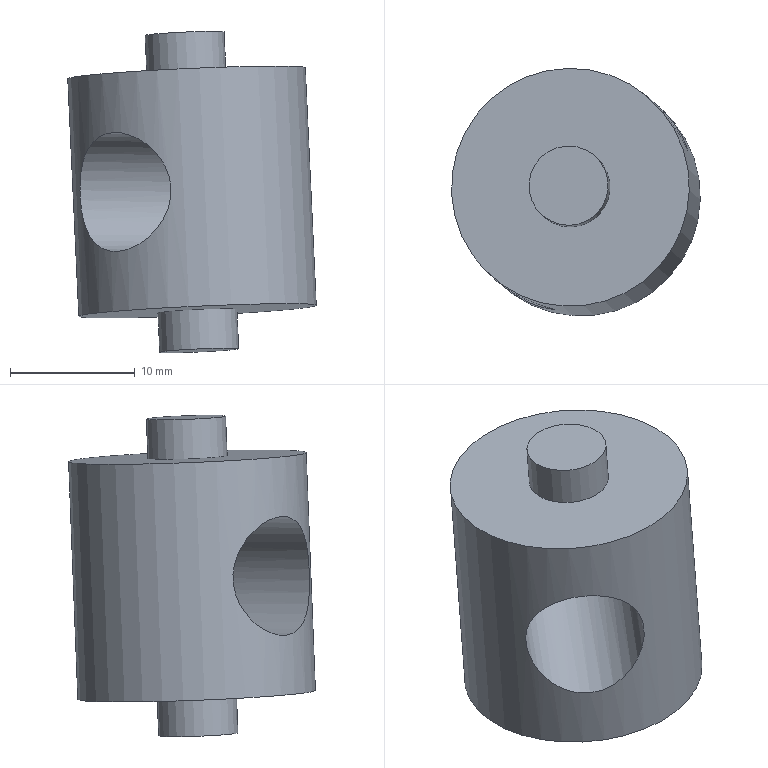Component | NX | ARTICULACION_A | 1 solid | 8 faces | box 19.91 x 19.77 x 25.74 mm | volume 4318 mm3 | cylinder 4 | plane 4 | commonest cylinder face diameters 6.35 x2 19.05 x1 9.525 x1
STEP:
#1=CARTESIAN_POINT('',(0.,0.,0.));
#2=DIRECTION('',(0.,0.,1.));
#3=DIRECTION('',(1.,0.,0.));
#4=AXIS2_PLACEMENT_3D('',#1,#2,#3);
#5=CARTESIAN_POINT('',(119.791,54.332,11.492));
#6=VERTEX_POINT('',#5);
#7=CARTESIAN_POINT('',(120.231,53.962,1.985));
#8=VERTEX_POINT('',#7);
#9=CARTESIAN_POINT('',(121.211,53.14,2.062));
#10=CARTESIAN_POINT('',(119.252,54.784,1.907));
#11=CARTESIAN_POINT('',(118.104,55.369,2.365));
#12=CARTESIAN_POINT('',(116.286,56.044,3.985));
#13=CARTESIAN_POINT('',(115.612,56.175,5.176));
#14=CARTESIAN_POINT('',(115.488,56.275,7.704));
#15=CARTESIAN_POINT('',(116.049,56.239,8.973));
#16=CARTESIAN_POINT('',(117.707,55.7,10.805));
#17=CARTESIAN_POINT('',(118.814,55.15,11.412));
#18=CARTESIAN_POINT('',(120.748,53.531,11.571));
#19=CARTESIAN_POINT('',(121.541,52.489,11.117));
#20=CARTESIAN_POINT('',(122.526,50.807,9.493));
#21=CARTESIAN_POINT('',(122.772,50.167,8.296));
#22=CARTESIAN_POINT('',(122.892,50.062,5.779));
#23=CARTESIAN_POINT('',(122.762,50.604,4.508));
#24=CARTESIAN_POINT('',(121.937,52.155,2.664));
#25=CARTESIAN_POINT('',(121.211,53.14,2.062));
#26=CARTESIAN_POINT('',(119.252,54.784,1.907));
#27=B_SPLINE_CURVE_WITH_KNOTS('',3,(#9,#10,#11,#12,#13,#14,#15,#16,#17,#18,#19,#20,#21,#22,#23,#24,#25,#26),.UNSPECIFIED.,.T.,.F.,(2,2,2,2,2,2,2,2,2,2,2),(-0.125,0.,0.125,0.25,0.375,0.5,0.625,0.75,0.875,1.,1.125),.UNSPECIFIED.);
#28=CARTESIAN_POINT('',(114.329,46.481,-2.769));
#29=DIRECTION('',(-0.04625,0.03881,0.9982));
#30=DIRECTION('',(0.6428,0.766,-0.));
#31=AXIS2_PLACEMENT_3D('',#28,#29,#30);
#32=CYLINDRICAL_SURFACE('',#31,9.525);
#33=CARTESIAN_POINT('',(6.283,4.763));
#34=CARTESIAN_POINT('',(6.308,4.763));
#35=CARTESIAN_POINT('',(6.356,4.798));
#36=CARTESIAN_POINT('',(6.427,4.949));
#37=CARTESIAN_POINT('',(6.495,5.191));
#38=CARTESIAN_POINT('',(6.559,5.518));
#39=CARTESIAN_POINT('',(6.619,5.92));
#40=CARTESIAN_POINT('',(6.671,6.392));
#41=CARTESIAN_POINT('',(6.717,6.931));
#42=CARTESIAN_POINT('',(6.755,7.523));
#43=CARTESIAN_POINT('',(6.784,8.159));
#44=CARTESIAN_POINT('',(6.802,8.825));
#45=CARTESIAN_POINT('',(6.809,9.514));
#46=CARTESIAN_POINT('',(6.803,10.203));
#47=CARTESIAN_POINT('',(6.784,10.873));
#48=CARTESIAN_POINT('',(6.756,11.513));
#49=CARTESIAN_POINT('',(6.718,12.11));
#50=CARTESIAN_POINT('',(6.672,12.652));
#51=CARTESIAN_POINT('',(6.619,13.125));
#52=CARTESIAN_POINT('',(6.56,13.528));
#53=CARTESIAN_POINT('',(6.496,13.855));
#54=CARTESIAN_POINT('',(6.427,14.098));
#55=CARTESIAN_POINT('',(6.357,14.251));
#56=CARTESIAN_POINT('',(6.285,14.305));
#57=CARTESIAN_POINT('',(6.212,14.254));
#58=CARTESIAN_POINT('',(6.141,14.104));
#59=CARTESIAN_POINT('',(6.073,13.863));
#60=CARTESIAN_POINT('',(6.008,13.537));
#61=CARTESIAN_POINT('',(5.948,13.134));
#62=CARTESIAN_POINT('',(5.895,12.661));
#63=CARTESIAN_POINT('',(5.849,12.12));
#64=CARTESIAN_POINT('',(5.811,11.526));
#65=CARTESIAN_POINT('',(5.782,10.889));
#66=CARTESIAN_POINT('',(5.764,10.223));
#67=CARTESIAN_POINT('',(5.757,9.537));
#68=CARTESIAN_POINT('',(5.764,8.85));
#69=CARTESIAN_POINT('',(5.782,8.181));
#70=CARTESIAN_POINT('',(5.81,7.541));
#71=CARTESIAN_POINT('',(5.848,6.942));
#72=CARTESIAN_POINT('',(5.894,6.398));
#73=CARTESIAN_POINT('',(5.948,5.922));
#74=CARTESIAN_POINT('',(6.007,5.517));
#75=CARTESIAN_POINT('',(6.071,5.19));
#76=CARTESIAN_POINT('',(6.139,4.948));
#77=CARTESIAN_POINT('',(6.21,4.797));
#78=CARTESIAN_POINT('',(6.259,4.763));
#79=CARTESIAN_POINT('',(6.283,4.763));
#80=B_SPLINE_CURVE_WITH_KNOTS('',3,(#33,#34,#35,#36,#37,#38,#39,#40,#41,#42,#43,#44,#45,#46,#47,#48,#49,#50,#51,#52,#53,#54,#55,#56,#57,#58,#59,#60,#61,#62,#63,#64,#65,#66,#67,#68,#69,#70,#71,#72,#73,#74,#75,#76,#77,#78,#79),.UNSPECIFIED.,.T.,.F.,(4,1,1,1,1,1,1,1,1,1,1,1,1,1,1,1,1,1,1,1,1,1,1,1,1,1,1,1,1,1,1,1,1,1,1,1,1,1,1,1,1,1,1,1,4),(0.,0.02273,0.04545,0.06818,0.09091,0.1136,0.1364,0.1591,0.1818,0.2045,0.2273,0.25,0.2727,0.2955,0.3182,0.3409,0.3636,0.3864,0.4091,0.4318,0.4545,0.4773,0.5,0.5227,0.5455,0.5682,0.5909,0.6136,0.6364,0.6591,0.6818,0.7045,0.7273,0.75,0.7727,0.7955,0.8182,0.8409,0.8636,0.8864,0.9091,0.9318,0.9545,0.9773,1.),.QUASI_UNIFORM_KNOTS.);
#81=(GEOMETRIC_REPRESENTATION_CONTEXT(2)PARAMETRIC_REPRESENTATION_CONTEXT()REPRESENTATION_CONTEXT('',''));
#82=DEFINITIONAL_REPRESENTATION('',(#80),#81);
#83=PCURVE('',#32,#82);
#84=CARTESIAN_POINT('',(106.052,37.511,6.738));
#85=DIRECTION('',(0.6428,0.766,0.));
#86=DIRECTION('',(0.04625,-0.03881,-0.9982));
#87=AXIS2_PLACEMENT_3D('',#84,#85,#86);
#88=CYLINDRICAL_SURFACE('',#87,4.763);
#89=CARTESIAN_POINT('',(3.142,21.717));
#90=CARTESIAN_POINT('',(3.19,21.717));
#91=CARTESIAN_POINT('',(3.286,21.698));
#92=CARTESIAN_POINT('',(3.43,21.621));
#93=CARTESIAN_POINT('',(3.574,21.504));
#94=CARTESIAN_POINT('',(3.717,21.358));
#95=CARTESIAN_POINT('',(3.858,21.19));
#96=CARTESIAN_POINT('',(3.998,21.01));
#97=CARTESIAN_POINT('',(4.14,20.835));
#98=CARTESIAN_POINT('',(4.282,20.678));
#99=CARTESIAN_POINT('',(4.424,20.55));
#100=CARTESIAN_POINT('',(4.567,20.463));
#101=CARTESIAN_POINT('',(4.711,20.43));
#102=CARTESIAN_POINT('',(4.855,20.463));
#103=CARTESIAN_POINT('',(4.999,20.549));
#104=CARTESIAN_POINT('',(5.142,20.677));
#105=CARTESIAN_POINT('',(5.285,20.835));
#106=CARTESIAN_POINT('',(5.427,21.01));
#107=CARTESIAN_POINT('',(5.567,21.191));
#108=CARTESIAN_POINT('',(5.709,21.359));
#109=CARTESIAN_POINT('',(5.851,21.505));
#110=CARTESIAN_POINT('',(5.993,21.621));
#111=CARTESIAN_POINT('',(6.137,21.698));
#112=CARTESIAN_POINT('',(6.234,21.717));
#113=CARTESIAN_POINT('',(6.283,21.717));
#114=B_SPLINE_CURVE_WITH_KNOTS('',3,(#89,#90,#91,#92,#93,#94,#95,#96,#97,#98,#99,#100,#101,#102,#103,#104,#105,#106,#107,#108,#109,#110,#111,#112,#113),.UNSPECIFIED.,.F.,.F.,(4,1,1,1,1,1,1,1,1,1,1,1,1,1,1,1,1,1,1,1,1,1,4),(0.5004,0.5231,0.5459,0.5686,0.5913,0.614,0.6367,0.6594,0.6821,0.7048,0.7275,0.7502,0.7729,0.7956,0.8183,0.841,0.8638,0.8865,0.9092,0.9319,0.9546,0.9773,1.),.QUASI_UNIFORM_KNOTS.);
#115=(GEOMETRIC_REPRESENTATION_CONTEXT(2)PARAMETRIC_REPRESENTATION_CONTEXT()REPRESENTATION_CONTEXT('',''));
#116=DEFINITIONAL_REPRESENTATION('',(#114),#115);
#117=PCURVE('',#88,#116);
#118=SURFACE_CURVE('',#27,(#83,#117),.PCURVE_S1.);
#119=EDGE_CURVE('',#6,#8,#118,.T.);
#120=ORIENTED_EDGE('',*,*,#119,.F.);
#121=CARTESIAN_POINT('',(119.571,54.517,16.246));
#122=VERTEX_POINT('',#121);
#123=CARTESIAN_POINT('',(119.791,54.332,11.492));
#124=CARTESIAN_POINT('',(119.571,54.517,16.246));
#125=B_SPLINE_CURVE_WITH_KNOTS('',1,(#123,#124),.UNSPECIFIED.,.F.,.F.,(2,2),(14.287,19.05),.PIECEWISE_BEZIER_KNOTS.);
#126=CARTESIAN_POINT('',(6.283,0.));
#127=DIRECTION('',(0.,1.));
#128=VECTOR('',#127,1.);
#129=LINE('',#126,#128);
#130=(GEOMETRIC_REPRESENTATION_CONTEXT(2)PARAMETRIC_REPRESENTATION_CONTEXT()REPRESENTATION_CONTEXT('',''));
#131=DEFINITIONAL_REPRESENTATION('',(#129),#130);
#132=PCURVE('',#32,#131);
#133=CARTESIAN_POINT('',(0.,0.));
#134=DIRECTION('',(0.,1.));
#135=VECTOR('',#134,1.);
#136=LINE('',#133,#135);
#137=(GEOMETRIC_REPRESENTATION_CONTEXT(2)PARAMETRIC_REPRESENTATION_CONTEXT()REPRESENTATION_CONTEXT('',''));
#138=DEFINITIONAL_REPRESENTATION('',(#136),#137);
#139=PCURVE('',#32,#138);
#140=SEAM_CURVE('',#125,(#132,#139),.PCURVE_S1.);
#141=EDGE_CURVE('',#6,#122,#140,.T.);
#142=ORIENTED_EDGE('',*,*,#141,.T.);
#143=CARTESIAN_POINT('',(113.448,47.22,16.246));
#144=DIRECTION('',(-0.04625,0.03881,0.9982));
#145=DIRECTION('',(0.6428,0.766,-0.));
#146=AXIS2_PLACEMENT_3D('',#143,#144,#145);
#147=CIRCLE('',#146,9.525);
#148=CARTESIAN_POINT('',(0.,19.05));
#149=DIRECTION('',(1.,0.));
#150=VECTOR('',#149,1.);
#151=LINE('',#148,#150);
#152=(GEOMETRIC_REPRESENTATION_CONTEXT(2)PARAMETRIC_REPRESENTATION_CONTEXT()REPRESENTATION_CONTEXT('',''));
#153=DEFINITIONAL_REPRESENTATION('',(#151),#152);
#154=PCURVE('',#32,#153);
#155=CARTESIAN_POINT('',(113.448,47.22,16.246));
#156=DIRECTION('',(-0.04625,0.03881,0.9982));
#157=DIRECTION('',(0.6428,0.766,-0.));
#158=AXIS2_PLACEMENT_3D('',#155,#156,#157);
#159=PLANE('',#158);
#160=CARTESIAN_POINT('',(0.,0.));
#161=DIRECTION('',(1.,0.));
#162=AXIS2_PLACEMENT_2D('',#160,#161);
#163=CIRCLE('',#162,9.525);
#164=(GEOMETRIC_REPRESENTATION_CONTEXT(2)PARAMETRIC_REPRESENTATION_CONTEXT()REPRESENTATION_CONTEXT('',''));
#165=DEFINITIONAL_REPRESENTATION('',(#163),#164);
#166=PCURVE('',#159,#165);
#167=SURFACE_CURVE('',#147,(#154,#166),.PCURVE_S1.);
#168=EDGE_CURVE('',#122,#122,#167,.T.);
#169=ORIENTED_EDGE('',*,*,#168,.F.);
#170=ORIENTED_EDGE('',*,*,#141,.F.);
#171=CARTESIAN_POINT('',(121.211,53.14,2.062));
#172=CARTESIAN_POINT('',(119.252,54.784,1.907));
#173=CARTESIAN_POINT('',(118.104,55.369,2.365));
#174=CARTESIAN_POINT('',(116.286,56.044,3.985));
#175=CARTESIAN_POINT('',(115.612,56.175,5.176));
#176=CARTESIAN_POINT('',(115.488,56.275,7.704));
#177=CARTESIAN_POINT('',(116.049,56.239,8.973));
#178=CARTESIAN_POINT('',(117.707,55.7,10.805));
#179=CARTESIAN_POINT('',(118.814,55.15,11.412));
#180=CARTESIAN_POINT('',(120.748,53.531,11.571));
#181=CARTESIAN_POINT('',(121.541,52.489,11.117));
#182=CARTESIAN_POINT('',(122.526,50.807,9.493));
#183=CARTESIAN_POINT('',(122.772,50.167,8.296));
#184=CARTESIAN_POINT('',(122.892,50.062,5.779));
#185=CARTESIAN_POINT('',(122.762,50.604,4.508));
#186=CARTESIAN_POINT('',(121.937,52.155,2.664));
#187=CARTESIAN_POINT('',(121.211,53.14,2.062));
#188=CARTESIAN_POINT('',(119.252,54.784,1.907));
#189=B_SPLINE_CURVE_WITH_KNOTS('',3,(#171,#172,#173,#174,#175,#176,#177,#178,#179,#180,#181,#182,#183,#184,#185,#186,#187,#188),.UNSPECIFIED.,.T.,.F.,(2,2,2,2,2,2,2,2,2,2,2),(-0.125,0.,0.125,0.25,0.375,0.5,0.625,0.75,0.875,1.,1.125),.UNSPECIFIED.);
#190=CARTESIAN_POINT('',(-0.,4.763));
#191=CARTESIAN_POINT('',(0.02444,4.763));
#192=CARTESIAN_POINT('',(0.07298,4.798));
#193=CARTESIAN_POINT('',(0.1439,4.949));
#194=CARTESIAN_POINT('',(0.212,5.191));
#195=CARTESIAN_POINT('',(0.2762,5.518));
#196=CARTESIAN_POINT('',(0.3354,5.92));
#197=CARTESIAN_POINT('',(0.3883,6.392));
#198=CARTESIAN_POINT('',(0.4342,6.931));
#199=CARTESIAN_POINT('',(0.4721,7.523));
#200=CARTESIAN_POINT('',(0.5008,8.159));
#201=CARTESIAN_POINT('',(0.5191,8.825));
#202=CARTESIAN_POINT('',(0.5258,9.514));
#203=CARTESIAN_POINT('',(0.5194,10.203));
#204=CARTESIAN_POINT('',(0.5013,10.873));
#205=CARTESIAN_POINT('',(0.4727,11.513));
#206=CARTESIAN_POINT('',(0.4348,12.11));
#207=CARTESIAN_POINT('',(0.3889,12.652));
#208=CARTESIAN_POINT('',(0.336,13.125));
#209=CARTESIAN_POINT('',(0.2767,13.528));
#210=CARTESIAN_POINT('',(0.2123,13.855));
#211=CARTESIAN_POINT('',(0.1442,14.098));
#212=CARTESIAN_POINT('',(0.07358,14.251));
#213=CARTESIAN_POINT('',(0.001407,14.305));
#214=CARTESIAN_POINT('',(-0.07088,14.254));
#215=CARTESIAN_POINT('',(-0.1418,14.104));
#216=CARTESIAN_POINT('',(-0.2103,13.863));
#217=CARTESIAN_POINT('',(-0.2751,13.537));
#218=CARTESIAN_POINT('',(-0.3348,13.134));
#219=CARTESIAN_POINT('',(-0.388,12.661));
#220=CARTESIAN_POINT('',(-0.4341,12.12));
#221=CARTESIAN_POINT('',(-0.4721,11.526));
#222=CARTESIAN_POINT('',(-0.5008,10.889));
#223=CARTESIAN_POINT('',(-0.5191,10.223));
#224=CARTESIAN_POINT('',(-0.5258,9.537));
#225=CARTESIAN_POINT('',(-0.5195,8.85));
#226=CARTESIAN_POINT('',(-0.5015,8.181));
#227=CARTESIAN_POINT('',(-0.4729,7.541));
#228=CARTESIAN_POINT('',(-0.435,6.942));
#229=CARTESIAN_POINT('',(-0.3889,6.398));
#230=CARTESIAN_POINT('',(-0.3356,5.922));
#231=CARTESIAN_POINT('',(-0.2762,5.517));
#232=CARTESIAN_POINT('',(-0.2119,5.19));
#233=CARTESIAN_POINT('',(-0.1438,4.948));
#234=CARTESIAN_POINT('',(-0.07297,4.797));
#235=CARTESIAN_POINT('',(-0.02444,4.763));
#236=CARTESIAN_POINT('',(-0.,4.763));
#237=B_SPLINE_CURVE_WITH_KNOTS('',3,(#190,#191,#192,#193,#194,#195,#196,#197,#198,#199,#200,#201,#202,#203,#204,#205,#206,#207,#208,#209,#210,#211,#212,#213,#214,#215,#216,#217,#218,#219,#220,#221,#222,#223,#224,#225,#226,#227,#228,#229,#230,#231,#232,#233,#234,#235,#236),.UNSPECIFIED.,.T.,.F.,(4,1,1,1,1,1,1,1,1,1,1,1,1,1,1,1,1,1,1,1,1,1,1,1,1,1,1,1,1,1,1,1,1,1,1,1,1,1,1,1,1,1,1,1,4),(0.,0.02273,0.04545,0.06818,0.09091,0.1136,0.1364,0.1591,0.1818,0.2045,0.2273,0.25,0.2727,0.2955,0.3182,0.3409,0.3636,0.3864,0.4091,0.4318,0.4545,0.4773,0.5,0.5227,0.5455,0.5682,0.5909,0.6136,0.6364,0.6591,0.6818,0.7045,0.7273,0.75,0.7727,0.7955,0.8182,0.8409,0.8636,0.8864,0.9091,0.9318,0.9545,0.9773,1.),.QUASI_UNIFORM_KNOTS.);
#238=(GEOMETRIC_REPRESENTATION_CONTEXT(2)PARAMETRIC_REPRESENTATION_CONTEXT()REPRESENTATION_CONTEXT('',''));
#239=DEFINITIONAL_REPRESENTATION('',(#237),#238);
#240=PCURVE('',#32,#239);
#241=CARTESIAN_POINT('',(0.,21.717));
#242=CARTESIAN_POINT('',(0.04891,21.717));
#243=CARTESIAN_POINT('',(0.1461,21.698));
#244=CARTESIAN_POINT('',(0.2904,21.621));
#245=CARTESIAN_POINT('',(0.4336,21.504));
#246=CARTESIAN_POINT('',(0.5757,21.358));
#247=CARTESIAN_POINT('',(0.7167,21.19));
#248=CARTESIAN_POINT('',(0.8564,21.011));
#249=CARTESIAN_POINT('',(0.9973,20.836));
#250=CARTESIAN_POINT('',(1.139,20.678));
#251=CARTESIAN_POINT('',(1.282,20.55));
#252=CARTESIAN_POINT('',(1.425,20.463));
#253=CARTESIAN_POINT('',(1.57,20.43));
#254=CARTESIAN_POINT('',(1.715,20.463));
#255=CARTESIAN_POINT('',(1.859,20.55));
#256=CARTESIAN_POINT('',(2.002,20.679));
#257=CARTESIAN_POINT('',(2.145,20.837));
#258=CARTESIAN_POINT('',(2.286,21.012));
#259=CARTESIAN_POINT('',(2.426,21.192));
#260=CARTESIAN_POINT('',(2.567,21.359));
#261=CARTESIAN_POINT('',(2.71,21.505));
#262=CARTESIAN_POINT('',(2.853,21.621));
#263=CARTESIAN_POINT('',(2.997,21.698));
#264=CARTESIAN_POINT('',(3.093,21.717));
#265=CARTESIAN_POINT('',(3.142,21.717));
#266=B_SPLINE_CURVE_WITH_KNOTS('',3,(#241,#242,#243,#244,#245,#246,#247,#248,#249,#250,#251,#252,#253,#254,#255,#256,#257,#258,#259,#260,#261,#262,#263,#264,#265),.UNSPECIFIED.,.F.,.F.,(4,1,1,1,1,1,1,1,1,1,1,1,1,1,1,1,1,1,1,1,1,1,4),(0.,0.02275,0.04549,0.06824,0.09099,0.1137,0.1365,0.1592,0.182,0.2047,0.2275,0.2502,0.273,0.2957,0.3185,0.3412,0.364,0.3867,0.4094,0.4322,0.4549,0.4777,0.5004),.QUASI_UNIFORM_KNOTS.);
#267=(GEOMETRIC_REPRESENTATION_CONTEXT(2)PARAMETRIC_REPRESENTATION_CONTEXT()REPRESENTATION_CONTEXT('',''));
#268=DEFINITIONAL_REPRESENTATION('',(#266),#267);
#269=PCURVE('',#88,#268);
#270=SURFACE_CURVE('',#189,(#240,#269),.PCURVE_S1.);
#271=EDGE_CURVE('',#8,#6,#270,.T.);
#272=ORIENTED_EDGE('',*,*,#271,.F.);
#273=CARTESIAN_POINT('',(120.452,53.778,-2.769));
#274=VERTEX_POINT('',#273);
#275=CARTESIAN_POINT('',(120.452,53.778,-2.769));
#276=CARTESIAN_POINT('',(120.231,53.962,1.985));
#277=B_SPLINE_CURVE_WITH_KNOTS('',1,(#275,#276),.UNSPECIFIED.,.F.,.F.,(2,2),(0.,4.763),.PIECEWISE_BEZIER_KNOTS.);
#278=CARTESIAN_POINT('',(0.,0.));
#279=DIRECTION('',(0.,1.));
#280=VECTOR('',#279,1.);
#281=LINE('',#278,#280);
#282=(GEOMETRIC_REPRESENTATION_CONTEXT(2)PARAMETRIC_REPRESENTATION_CONTEXT()REPRESENTATION_CONTEXT('',''));
#283=DEFINITIONAL_REPRESENTATION('',(#281),#282);
#284=PCURVE('',#32,#283);
#285=CARTESIAN_POINT('',(6.283,0.));
#286=DIRECTION('',(0.,1.));
#287=VECTOR('',#286,1.);
#288=LINE('',#285,#287);
#289=(GEOMETRIC_REPRESENTATION_CONTEXT(2)PARAMETRIC_REPRESENTATION_CONTEXT()REPRESENTATION_CONTEXT('',''));
#290=DEFINITIONAL_REPRESENTATION('',(#288),#289);
#291=PCURVE('',#32,#290);
#292=SEAM_CURVE('',#277,(#284,#291),.PCURVE_S1.);
#293=EDGE_CURVE('',#274,#8,#292,.T.);
#294=ORIENTED_EDGE('',*,*,#293,.F.);
#295=CARTESIAN_POINT('',(114.329,46.481,-2.769));
#296=DIRECTION('',(-0.04625,0.03881,0.9982));
#297=DIRECTION('',(0.6428,0.766,-0.));
#298=AXIS2_PLACEMENT_3D('',#295,#296,#297);
#299=CIRCLE('',#298,9.525);
#300=CARTESIAN_POINT('',(0.,0.));
#301=DIRECTION('',(1.,0.));
#302=VECTOR('',#301,1.);
#303=LINE('',#300,#302);
#304=(GEOMETRIC_REPRESENTATION_CONTEXT(2)PARAMETRIC_REPRESENTATION_CONTEXT()REPRESENTATION_CONTEXT('',''));
#305=DEFINITIONAL_REPRESENTATION('',(#303),#304);
#306=PCURVE('',#32,#305);
#307=CARTESIAN_POINT('',(114.329,46.481,-2.769));
#308=DIRECTION('',(-0.04625,0.03881,0.9982));
#309=DIRECTION('',(0.6428,0.766,-0.));
#310=AXIS2_PLACEMENT_3D('',#307,#308,#309);
#311=PLANE('',#310);
#312=CARTESIAN_POINT('',(0.,0.));
#313=DIRECTION('',(1.,0.));
#314=AXIS2_PLACEMENT_2D('',#312,#313);
#315=CIRCLE('',#314,9.525);
#316=(GEOMETRIC_REPRESENTATION_CONTEXT(2)PARAMETRIC_REPRESENTATION_CONTEXT()REPRESENTATION_CONTEXT('',''));
#317=DEFINITIONAL_REPRESENTATION('',(#315),#316);
#318=PCURVE('',#311,#317);
#319=SURFACE_CURVE('',#299,(#306,#318),.PCURVE_S1.);
#320=EDGE_CURVE('',#274,#274,#319,.T.);
#321=ORIENTED_EDGE('',*,*,#320,.T.);
#322=ORIENTED_EDGE('',*,*,#293,.T.);
#323=EDGE_LOOP('',(#120,#142,#169,#170,#272,#294,#321,#322));
#324=FACE_BOUND('',#323,.T.);
#325=CARTESIAN_POINT('',(107.986,39.369,1.985));
#326=VERTEX_POINT('',#325);
#327=CARTESIAN_POINT('',(107.007,40.191,1.907));
#328=CARTESIAN_POINT('',(108.966,38.547,2.062));
#329=CARTESIAN_POINT('',(110.064,38.003,2.668));
#330=CARTESIAN_POINT('',(111.723,37.463,4.496));
#331=CARTESIAN_POINT('',(112.284,37.427,5.75));
#332=CARTESIAN_POINT('',(112.173,37.524,8.279));
#333=CARTESIAN_POINT('',(111.497,37.656,9.485));
#334=CARTESIAN_POINT('',(109.679,38.329,11.108));
#335=CARTESIAN_POINT('',(108.523,38.921,11.566));
#336=CARTESIAN_POINT('',(106.588,40.54,11.42));
#337=CARTESIAN_POINT('',(105.844,41.541,10.816));
#338=CARTESIAN_POINT('',(105.019,43.088,8.982));
#339=CARTESIAN_POINT('',(104.887,43.633,7.722));
#340=CARTESIAN_POINT('',(105.001,43.542,5.204));
#341=CARTESIAN_POINT('',(105.246,42.904,3.996));
#342=CARTESIAN_POINT('',(106.232,41.217,2.361));
#343=CARTESIAN_POINT('',(107.007,40.191,1.907));
#344=CARTESIAN_POINT('',(108.966,38.547,2.062));
#345=B_SPLINE_CURVE_WITH_KNOTS('',3,(#327,#328,#329,#330,#331,#332,#333,#334,#335,#336,#337,#338,#339,#340,#341,#342,#343,#344),.UNSPECIFIED.,.T.,.F.,(2,2,2,2,2,2,2,2,2,2,2),(-0.125,0.,0.125,0.25,0.375,0.5,0.625,0.75,0.875,1.,1.125),.UNSPECIFIED.);
#346=CARTESIAN_POINT('',(3.142,4.763));
#347=CARTESIAN_POINT('',(3.166,4.763));
#348=CARTESIAN_POINT('',(3.215,4.798));
#349=CARTESIAN_POINT('',(3.285,4.949));
#350=CARTESIAN_POINT('',(3.354,5.191));
#351=CARTESIAN_POINT('',(3.418,5.518));
#352=CARTESIAN_POINT('',(3.477,5.92));
#353=CARTESIAN_POINT('',(3.53,6.392));
#354=CARTESIAN_POINT('',(3.576,6.931));
#355=CARTESIAN_POINT('',(3.614,7.523));
#356=CARTESIAN_POINT('',(3.642,8.159));
#357=CARTESIAN_POINT('',(3.661,8.825));
#358=CARTESIAN_POINT('',(3.667,9.514));
#359=CARTESIAN_POINT('',(3.661,10.203));
#360=CARTESIAN_POINT('',(3.643,10.873));
#361=CARTESIAN_POINT('',(3.614,11.513));
#362=CARTESIAN_POINT('',(3.576,12.11));
#363=CARTESIAN_POINT('',(3.53,12.652));
#364=CARTESIAN_POINT('',(3.478,13.125));
#365=CARTESIAN_POINT('',(3.418,13.528));
#366=CARTESIAN_POINT('',(3.354,13.855));
#367=CARTESIAN_POINT('',(3.286,14.098));
#368=CARTESIAN_POINT('',(3.215,14.251));
#369=CARTESIAN_POINT('',(3.143,14.305));
#370=CARTESIAN_POINT('',(3.071,14.254));
#371=CARTESIAN_POINT('',(3.,14.104));
#372=CARTESIAN_POINT('',(2.931,13.863));
#373=CARTESIAN_POINT('',(2.866,13.537));
#374=CARTESIAN_POINT('',(2.807,13.134));
#375=CARTESIAN_POINT('',(2.754,12.661));
#376=CARTESIAN_POINT('',(2.707,12.12));
#377=CARTESIAN_POINT('',(2.67,11.526));
#378=CARTESIAN_POINT('',(2.641,10.889));
#379=CARTESIAN_POINT('',(2.622,10.223));
#380=CARTESIAN_POINT('',(2.616,9.537));
#381=CARTESIAN_POINT('',(2.622,8.85));
#382=CARTESIAN_POINT('',(2.64,8.181));
#383=CARTESIAN_POINT('',(2.669,7.541));
#384=CARTESIAN_POINT('',(2.707,6.942));
#385=CARTESIAN_POINT('',(2.753,6.398));
#386=CARTESIAN_POINT('',(2.806,5.922));
#387=CARTESIAN_POINT('',(2.865,5.517));
#388=CARTESIAN_POINT('',(2.93,5.19));
#389=CARTESIAN_POINT('',(2.998,4.948));
#390=CARTESIAN_POINT('',(3.069,4.797));
#391=CARTESIAN_POINT('',(3.117,4.763));
#392=CARTESIAN_POINT('',(3.142,4.763));
#393=B_SPLINE_CURVE_WITH_KNOTS('',3,(#346,#347,#348,#349,#350,#351,#352,#353,#354,#355,#356,#357,#358,#359,#360,#361,#362,#363,#364,#365,#366,#367,#368,#369,#370,#371,#372,#373,#374,#375,#376,#377,#378,#379,#380,#381,#382,#383,#384,#385,#386,#387,#388,#389,#390,#391,#392),.UNSPECIFIED.,.T.,.F.,(4,1,1,1,1,1,1,1,1,1,1,1,1,1,1,1,1,1,1,1,1,1,1,1,1,1,1,1,1,1,1,1,1,1,1,1,1,1,1,1,1,1,1,1,4),(0.,0.02273,0.04545,0.06818,0.09091,0.1136,0.1364,0.1591,0.1818,0.2045,0.2273,0.25,0.2727,0.2955,0.3182,0.3409,0.3636,0.3864,0.4091,0.4318,0.4545,0.4773,0.5,0.5227,0.5455,0.5682,0.5909,0.6136,0.6364,0.6591,0.6818,0.7045,0.7273,0.75,0.7727,0.7955,0.8182,0.8409,0.8636,0.8864,0.9091,0.9318,0.9545,0.9773,1.),.QUASI_UNIFORM_KNOTS.);
#394=(GEOMETRIC_REPRESENTATION_CONTEXT(2)PARAMETRIC_REPRESENTATION_CONTEXT()REPRESENTATION_CONTEXT('',''));
#395=DEFINITIONAL_REPRESENTATION('',(#393),#394);
#396=PCURVE('',#32,#395);
#397=CARTESIAN_POINT('',(6.283,2.667));
#398=CARTESIAN_POINT('',(6.234,2.667));
#399=CARTESIAN_POINT('',(6.137,2.686));
#400=CARTESIAN_POINT('',(5.993,2.763));
#401=CARTESIAN_POINT('',(5.85,2.879));
#402=CARTESIAN_POINT('',(5.708,3.026));
#403=CARTESIAN_POINT('',(5.567,3.193));
#404=CARTESIAN_POINT('',(5.428,3.372));
#405=CARTESIAN_POINT('',(5.287,3.547));
#406=CARTESIAN_POINT('',(5.145,3.705));
#407=CARTESIAN_POINT('',(5.003,3.833));
#408=CARTESIAN_POINT('',(4.859,3.92));
#409=CARTESIAN_POINT('',(4.715,3.954));
#410=CARTESIAN_POINT('',(4.57,3.922));
#411=CARTESIAN_POINT('',(4.426,3.835));
#412=CARTESIAN_POINT('',(4.283,3.707));
#413=CARTESIAN_POINT('',(4.14,3.549));
#414=CARTESIAN_POINT('',(3.999,3.375));
#415=CARTESIAN_POINT('',(3.859,3.195));
#416=CARTESIAN_POINT('',(3.718,3.028));
#417=CARTESIAN_POINT('',(3.576,2.881));
#418=CARTESIAN_POINT('',(3.432,2.765));
#419=CARTESIAN_POINT('',(3.289,2.687));
#420=CARTESIAN_POINT('',(3.144,2.657));
#421=CARTESIAN_POINT('',(3.,2.685));
#422=CARTESIAN_POINT('',(2.856,2.762));
#423=CARTESIAN_POINT('',(2.712,2.877));
#424=CARTESIAN_POINT('',(2.569,3.024));
#425=CARTESIAN_POINT('',(2.427,3.191));
#426=CARTESIAN_POINT('',(2.287,3.371));
#427=CARTESIAN_POINT('',(2.145,3.546));
#428=CARTESIAN_POINT('',(2.003,3.704));
#429=CARTESIAN_POINT('',(1.861,3.833));
#430=CARTESIAN_POINT('',(1.717,3.92));
#431=CARTESIAN_POINT('',(1.573,3.954));
#432=CARTESIAN_POINT('',(1.429,3.922));
#433=CARTESIAN_POINT('',(1.285,3.836));
#434=CARTESIAN_POINT('',(1.142,3.708));
#435=CARTESIAN_POINT('',(0.9992,3.55));
#436=CARTESIAN_POINT('',(0.8574,3.375));
#437=CARTESIAN_POINT('',(0.7166,3.193));
#438=CARTESIAN_POINT('',(0.5752,3.026));
#439=CARTESIAN_POINT('',(0.433,2.879));
#440=CARTESIAN_POINT('',(0.29,2.763));
#441=CARTESIAN_POINT('',(0.1459,2.686));
#442=CARTESIAN_POINT('',(0.04887,2.667));
#443=CARTESIAN_POINT('',(-0.,2.667));
#444=B_SPLINE_CURVE_WITH_KNOTS('',3,(#397,#398,#399,#400,#401,#402,#403,#404,#405,#406,#407,#408,#409,#410,#411,#412,#413,#414,#415,#416,#417,#418,#419,#420,#421,#422,#423,#424,#425,#426,#427,#428,#429,#430,#431,#432,#433,#434,#435,#436,#437,#438,#439,#440,#441,#442,#443),.UNSPECIFIED.,.F.,.F.,(4,1,1,1,1,1,1,1,1,1,1,1,1,1,1,1,1,1,1,1,1,1,1,1,1,1,1,1,1,1,1,1,1,1,1,1,1,1,1,1,1,1,1,1,4),(0.,0.02273,0.04545,0.06818,0.09091,0.1136,0.1364,0.1591,0.1818,0.2045,0.2273,0.25,0.2727,0.2955,0.3182,0.3409,0.3636,0.3864,0.4091,0.4318,0.4545,0.4773,0.5,0.5227,0.5455,0.5682,0.5909,0.6136,0.6364,0.6591,0.6818,0.7045,0.7273,0.75,0.7727,0.7955,0.8182,0.8409,0.8636,0.8864,0.9091,0.9318,0.9545,0.9773,1.),.QUASI_UNIFORM_KNOTS.);
#445=(GEOMETRIC_REPRESENTATION_CONTEXT(2)PARAMETRIC_REPRESENTATION_CONTEXT()REPRESENTATION_CONTEXT('',''));
#446=DEFINITIONAL_REPRESENTATION('',(#444),#445);
#447=PCURVE('',#88,#446);
#448=SURFACE_CURVE('',#345,(#396,#447),.PCURVE_S1.);
#449=EDGE_CURVE('',#326,#326,#448,.T.);
#450=ORIENTED_EDGE('',*,*,#449,.F.);
#451=EDGE_LOOP('',(#450));
#452=FACE_BOUND('',#451,.T.);
#453=ADVANCED_FACE('',(#324,#452),#32,.T.);
#454=CARTESIAN_POINT('',(116.37,48.913,-2.769));
#455=VERTEX_POINT('',#454);
#456=CARTESIAN_POINT('',(114.329,46.481,-2.769));
#457=DIRECTION('',(-0.04625,0.03881,0.9982));
#458=DIRECTION('',(0.6428,0.766,0.));
#459=AXIS2_PLACEMENT_3D('',#456,#457,#458);
#460=CIRCLE('',#459,3.175);
#461=CARTESIAN_POINT('',(0.,0.));
#462=DIRECTION('',(1.,-0.));
#463=AXIS2_PLACEMENT_2D('',#461,#462);
#464=CIRCLE('',#463,3.175);
#465=(GEOMETRIC_REPRESENTATION_CONTEXT(2)PARAMETRIC_REPRESENTATION_CONTEXT()REPRESENTATION_CONTEXT('',''));
#466=DEFINITIONAL_REPRESENTATION('',(#464),#465);
#467=PCURVE('',#311,#466);
#468=CARTESIAN_POINT('',(114.476,46.358,-5.938));
#469=DIRECTION('',(-0.04625,0.03881,0.9982));
#470=DIRECTION('',(0.6428,0.766,0.));
#471=AXIS2_PLACEMENT_3D('',#468,#469,#470);
#472=CYLINDRICAL_SURFACE('',#471,3.175);
#473=CARTESIAN_POINT('',(0.,3.175));
#474=DIRECTION('',(1.,0.));
#475=VECTOR('',#474,1.);
#476=LINE('',#473,#475);
#477=(GEOMETRIC_REPRESENTATION_CONTEXT(2)PARAMETRIC_REPRESENTATION_CONTEXT()REPRESENTATION_CONTEXT('',''));
#478=DEFINITIONAL_REPRESENTATION('',(#476),#477);
#479=PCURVE('',#472,#478);
#480=SURFACE_CURVE('',#460,(#467,#479),.PCURVE_S1.);
#481=EDGE_CURVE('',#455,#455,#480,.T.);
#482=ORIENTED_EDGE('',*,*,#481,.T.);
#483=EDGE_LOOP('',(#482));
#484=FACE_BOUND('',#483,.T.);
#485=ORIENTED_EDGE('',*,*,#320,.F.);
#486=EDGE_LOOP('',(#485));
#487=FACE_BOUND('',#486,.T.);
#488=ADVANCED_FACE('',(#484,#487),#311,.F.);
#489=CARTESIAN_POINT('',(115.489,49.652,16.246));
#490=VERTEX_POINT('',#489);
#491=CARTESIAN_POINT('',(113.448,47.22,16.246));
#492=DIRECTION('',(-0.04625,0.03881,0.9982));
#493=DIRECTION('',(0.6428,0.766,0.));
#494=AXIS2_PLACEMENT_3D('',#491,#492,#493);
#495=CIRCLE('',#494,3.175);
#496=CARTESIAN_POINT('',(0.,0.));
#497=DIRECTION('',(1.,-0.));
#498=AXIS2_PLACEMENT_2D('',#496,#497);
#499=CIRCLE('',#498,3.175);
#500=(GEOMETRIC_REPRESENTATION_CONTEXT(2)PARAMETRIC_REPRESENTATION_CONTEXT()REPRESENTATION_CONTEXT('',''));
#501=DEFINITIONAL_REPRESENTATION('',(#499),#500);
#502=PCURVE('',#159,#501);
#503=CARTESIAN_POINT('',(114.476,46.358,-5.938));
#504=DIRECTION('',(-0.04625,0.03881,0.9982));
#505=DIRECTION('',(0.6428,0.766,0.));
#506=AXIS2_PLACEMENT_3D('',#503,#504,#505);
#507=CYLINDRICAL_SURFACE('',#506,3.175);
#508=CARTESIAN_POINT('',(0.,22.225));
#509=DIRECTION('',(1.,0.));
#510=VECTOR('',#509,1.);
#511=LINE('',#508,#510);
#512=(GEOMETRIC_REPRESENTATION_CONTEXT(2)PARAMETRIC_REPRESENTATION_CONTEXT()REPRESENTATION_CONTEXT('',''));
#513=DEFINITIONAL_REPRESENTATION('',(#511),#512);
#514=PCURVE('',#507,#513);
#515=SURFACE_CURVE('',#495,(#502,#514),.PCURVE_S1.);
#516=EDGE_CURVE('',#490,#490,#515,.T.);
#517=ORIENTED_EDGE('',*,*,#516,.F.);
#518=EDGE_LOOP('',(#517));
#519=FACE_BOUND('',#518,.T.);
#520=ORIENTED_EDGE('',*,*,#168,.T.);
#521=EDGE_LOOP('',(#520));
#522=FACE_BOUND('',#521,.T.);
#523=ADVANCED_FACE('',(#519,#522),#159,.T.);
#524=CARTESIAN_POINT('',(115.342,49.776,19.415));
#525=VERTEX_POINT('',#524);
#526=CARTESIAN_POINT('',(113.301,47.343,19.415));
#527=DIRECTION('',(-0.04625,0.03881,0.9982));
#528=DIRECTION('',(0.6428,0.766,0.));
#529=AXIS2_PLACEMENT_3D('',#526,#527,#528);
#530=CIRCLE('',#529,3.175);
#531=CARTESIAN_POINT('',(113.301,47.343,19.415));
#532=DIRECTION('',(-0.04625,0.03881,0.9982));
#533=DIRECTION('',(0.6428,0.766,0.));
#534=AXIS2_PLACEMENT_3D('',#531,#532,#533);
#535=PLANE('',#534);
#536=CARTESIAN_POINT('',(0.,0.));
#537=DIRECTION('',(1.,-0.));
#538=AXIS2_PLACEMENT_2D('',#536,#537);
#539=CIRCLE('',#538,3.175);
#540=(GEOMETRIC_REPRESENTATION_CONTEXT(2)PARAMETRIC_REPRESENTATION_CONTEXT()REPRESENTATION_CONTEXT('',''));
#541=DEFINITIONAL_REPRESENTATION('',(#539),#540);
#542=PCURVE('',#535,#541);
#543=CARTESIAN_POINT('',(0.,25.4));
#544=DIRECTION('',(1.,0.));
#545=VECTOR('',#544,1.);
#546=LINE('',#543,#545);
#547=(GEOMETRIC_REPRESENTATION_CONTEXT(2)PARAMETRIC_REPRESENTATION_CONTEXT()REPRESENTATION_CONTEXT('',''));
#548=DEFINITIONAL_REPRESENTATION('',(#546),#547);
#549=PCURVE('',#507,#548);
#550=SURFACE_CURVE('',#530,(#542,#549),.PCURVE_S1.);
#551=EDGE_CURVE('',#525,#525,#550,.T.);
#552=ORIENTED_EDGE('',*,*,#551,.T.);
#553=EDGE_LOOP('',(#552));
#554=FACE_BOUND('',#553,.T.);
#555=ADVANCED_FACE('',(#554),#535,.T.);
#556=ORIENTED_EDGE('',*,*,#516,.T.);
#557=CARTESIAN_POINT('',(115.489,49.652,16.246));
#558=CARTESIAN_POINT('',(115.342,49.776,19.415));
#559=B_SPLINE_CURVE_WITH_KNOTS('',1,(#557,#558),.UNSPECIFIED.,.F.,.F.,(2,2),(22.225,25.4),.PIECEWISE_BEZIER_KNOTS.);
#560=CARTESIAN_POINT('',(6.283,0.));
#561=DIRECTION('',(0.,1.));
#562=VECTOR('',#561,1.);
#563=LINE('',#560,#562);
#564=(GEOMETRIC_REPRESENTATION_CONTEXT(2)PARAMETRIC_REPRESENTATION_CONTEXT()REPRESENTATION_CONTEXT('',''));
#565=DEFINITIONAL_REPRESENTATION('',(#563),#564);
#566=PCURVE('',#507,#565);
#567=CARTESIAN_POINT('',(0.,0.));
#568=DIRECTION('',(0.,1.));
#569=VECTOR('',#568,1.);
#570=LINE('',#567,#569);
#571=(GEOMETRIC_REPRESENTATION_CONTEXT(2)PARAMETRIC_REPRESENTATION_CONTEXT()REPRESENTATION_CONTEXT('',''));
#572=DEFINITIONAL_REPRESENTATION('',(#570),#571);
#573=PCURVE('',#507,#572);
#574=SEAM_CURVE('',#559,(#566,#573),.PCURVE_S1.);
#575=EDGE_CURVE('',#490,#525,#574,.T.);
#576=ORIENTED_EDGE('',*,*,#575,.T.);
#577=ORIENTED_EDGE('',*,*,#551,.F.);
#578=ORIENTED_EDGE('',*,*,#575,.F.);
#579=EDGE_LOOP('',(#556,#576,#577,#578));
#580=FACE_BOUND('',#579,.T.);
#581=ADVANCED_FACE('',(#580),#507,.T.);
#582=CARTESIAN_POINT('',(116.517,48.79,-5.938));
#583=VERTEX_POINT('',#582);
#584=CARTESIAN_POINT('',(114.476,46.358,-5.938));
#585=DIRECTION('',(-0.04625,0.03881,0.9982));
#586=DIRECTION('',(0.6428,0.766,0.));
#587=AXIS2_PLACEMENT_3D('',#584,#585,#586);
#588=CIRCLE('',#587,3.175);
#589=CARTESIAN_POINT('',(0.,-0.));
#590=DIRECTION('',(1.,0.));
#591=VECTOR('',#590,1.);
#592=LINE('',#589,#591);
#593=(GEOMETRIC_REPRESENTATION_CONTEXT(2)PARAMETRIC_REPRESENTATION_CONTEXT()REPRESENTATION_CONTEXT('',''));
#594=DEFINITIONAL_REPRESENTATION('',(#592),#593);
#595=PCURVE('',#472,#594);
#596=CARTESIAN_POINT('',(114.476,46.358,-5.938));
#597=DIRECTION('',(-0.04625,0.03881,0.9982));
#598=DIRECTION('',(0.6428,0.766,-0.));
#599=AXIS2_PLACEMENT_3D('',#596,#597,#598);
#600=PLANE('',#599);
#601=CARTESIAN_POINT('',(0.,0.));
#602=DIRECTION('',(1.,-0.));
#603=AXIS2_PLACEMENT_2D('',#601,#602);
#604=CIRCLE('',#603,3.175);
#605=(GEOMETRIC_REPRESENTATION_CONTEXT(2)PARAMETRIC_REPRESENTATION_CONTEXT()REPRESENTATION_CONTEXT('',''));
#606=DEFINITIONAL_REPRESENTATION('',(#604),#605);
#607=PCURVE('',#600,#606);
#608=SURFACE_CURVE('',#588,(#595,#607),.PCURVE_S1.);
#609=EDGE_CURVE('',#583,#583,#608,.T.);
#610=ORIENTED_EDGE('',*,*,#609,.T.);
#611=CARTESIAN_POINT('',(116.517,48.79,-5.938));
#612=CARTESIAN_POINT('',(116.37,48.913,-2.769));
#613=B_SPLINE_CURVE_WITH_KNOTS('',1,(#611,#612),.UNSPECIFIED.,.F.,.F.,(2,2),(-0.,3.175),.PIECEWISE_BEZIER_KNOTS.);
#614=CARTESIAN_POINT('',(6.283,0.));
#615=DIRECTION('',(0.,1.));
#616=VECTOR('',#615,1.);
#617=LINE('',#614,#616);
#618=(GEOMETRIC_REPRESENTATION_CONTEXT(2)PARAMETRIC_REPRESENTATION_CONTEXT()REPRESENTATION_CONTEXT('',''));
#619=DEFINITIONAL_REPRESENTATION('',(#617),#618);
#620=PCURVE('',#472,#619);
#621=CARTESIAN_POINT('',(0.,0.));
#622=DIRECTION('',(0.,1.));
#623=VECTOR('',#622,1.);
#624=LINE('',#621,#623);
#625=(GEOMETRIC_REPRESENTATION_CONTEXT(2)PARAMETRIC_REPRESENTATION_CONTEXT()REPRESENTATION_CONTEXT('',''));
#626=DEFINITIONAL_REPRESENTATION('',(#624),#625);
#627=PCURVE('',#472,#626);
#628=SEAM_CURVE('',#613,(#620,#627),.PCURVE_S1.);
#629=EDGE_CURVE('',#583,#455,#628,.T.);
#630=ORIENTED_EDGE('',*,*,#629,.T.);
#631=ORIENTED_EDGE('',*,*,#481,.F.);
#632=ORIENTED_EDGE('',*,*,#629,.F.);
#633=EDGE_LOOP('',(#610,#630,#631,#632));
#634=FACE_BOUND('',#633,.T.);
#635=ADVANCED_FACE('',(#634),#472,.T.);
#636=ORIENTED_EDGE('',*,*,#609,.F.);
#637=EDGE_LOOP('',(#636));
#638=FACE_BOUND('',#637,.T.);
#639=ADVANCED_FACE('',(#638),#600,.F.);
#640=ORIENTED_EDGE('',*,*,#119,.F.);
#641=ORIENTED_EDGE('',*,*,#271,.F.);
#642=CARTESIAN_POINT('',(107.986,39.369,1.985));
#643=CARTESIAN_POINT('',(120.231,53.962,1.985));
#644=B_SPLINE_CURVE_WITH_KNOTS('',1,(#642,#643),.UNSPECIFIED.,.F.,.F.,(2,2),(2.667,21.717),.PIECEWISE_BEZIER_KNOTS.);
#645=CARTESIAN_POINT('',(0.,0.));
#646=DIRECTION('',(0.,1.));
#647=VECTOR('',#646,1.);
#648=LINE('',#645,#647);
#649=(GEOMETRIC_REPRESENTATION_CONTEXT(2)PARAMETRIC_REPRESENTATION_CONTEXT()REPRESENTATION_CONTEXT('',''));
#650=DEFINITIONAL_REPRESENTATION('',(#648),#649);
#651=PCURVE('',#88,#650);
#652=CARTESIAN_POINT('',(6.283,0.));
#653=DIRECTION('',(0.,1.));
#654=VECTOR('',#653,1.);
#655=LINE('',#652,#654);
#656=(GEOMETRIC_REPRESENTATION_CONTEXT(2)PARAMETRIC_REPRESENTATION_CONTEXT()REPRESENTATION_CONTEXT('',''));
#657=DEFINITIONAL_REPRESENTATION('',(#655),#656);
#658=PCURVE('',#88,#657);
#659=SEAM_CURVE('',#644,(#651,#658),.PCURVE_S1.);
#660=EDGE_CURVE('',#326,#8,#659,.T.);
#661=ORIENTED_EDGE('',*,*,#660,.F.);
#662=ORIENTED_EDGE('',*,*,#449,.F.);
#663=ORIENTED_EDGE('',*,*,#660,.T.);
#664=EDGE_LOOP('',(#640,#641,#661,#662,#663));
#665=FACE_BOUND('',#664,.F.);
#666=ADVANCED_FACE('',(#665),#88,.F.);
#667=CLOSED_SHELL('',(#453,#488,#523,#555,#581,#635,#639,#666));
#668=MANIFOLD_SOLID_BREP('',#667);
#669=(LENGTH_UNIT()NAMED_UNIT(*)SI_UNIT(.MILLI.,.METRE.));
#670=UNCERTAINTY_MEASURE_WITH_UNIT(LENGTH_MEASURE(0.002),#669,'','');
#671=(NAMED_UNIT(*)PLANE_ANGLE_UNIT()SI_UNIT($,.RADIAN.));
#672=(NAMED_UNIT(*)SI_UNIT($,.STERADIAN.)SOLID_ANGLE_UNIT());
#673=(GEOMETRIC_REPRESENTATION_CONTEXT(3)GLOBAL_UNCERTAINTY_ASSIGNED_CONTEXT((#670))GLOBAL_UNIT_ASSIGNED_CONTEXT((#669,#671,#672))REPRESENTATION_CONTEXT('',''));
#674=ADVANCED_BREP_SHAPE_REPRESENTATION('',(#4,#668),#673);